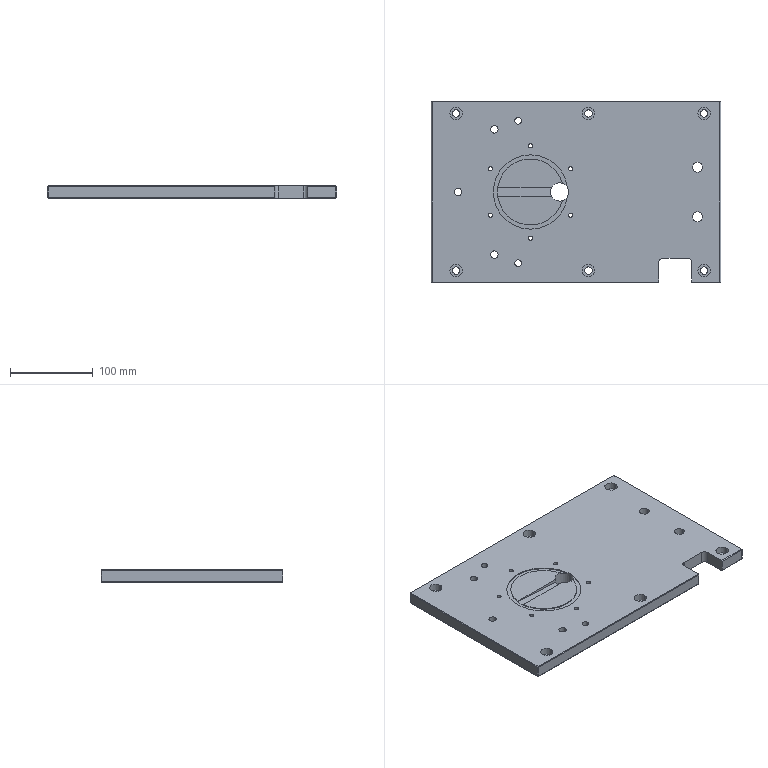Component | SolidWorks | ZN-A-008-1 | 1 solid | 110 faces | box 350 x 220 x 15 mm | volume 1103345 mm3 | cylinder 63 | plane 47 | commonest cylinder face diameters 15 x18 9 x18 5 x12 12 x4 8 x4 22 x2 80 x2 10 x2
build123d program:
from build123d import *

# Parameters (mm, degrees)
SKETCH1_W                                       = 350
SKETCH1_H                                       = 220
BOSS_EXTRUDE1_DEPTH                             = 15
F_8_0_8_DIAMETER_HOLE1_D                        = 8
F_8_0_8_DIAMETER_HOLE1_DEPTH                    = 15
F_8_0_8_DIAMETER_HOLE1_TIP                      = 2.403
M8_HEX_SOCKET_HEAD_CAP_SCREW_CBORE1_D           = 9
M8_HEX_SOCKET_HEAD_CAP_SCREW_CBORE1_CBORE_D     = 15
M8_HEX_SOCKET_HEAD_CAP_SCREW_CBORE1_CBORE_DEPTH = 8.6
M12_TAPPED_HOLE1_D                              = 12
M12_TAPPED_HOLE1_DEPTH                          = 29.25
M12_TAPPED_HOLE1_TIP                            = 3.605
M8_HEX_SOCKET_HEAD_CAP_SCREW_CBORE2_D           = 9
M8_HEX_SOCKET_HEAD_CAP_SCREW_CBORE2_CBORE_D     = 15
M8_HEX_SOCKET_HEAD_CAP_SCREW_CBORE2_CBORE_DEPTH = 8.6
CUT_EXTRUDE2_DEPTH                              = 50
CHAMFER2_SIZE                                   = 1
SKETCH12_R                                      = 11
CUT_EXTRUDE3_DEPTH                              = 90
SKETCH14_R                                      = 45
SKETCH14_R_2                                    = 40
CUT_EXTRUDE7_DEPTH                              = 1
CUT_EXTRUDE6_DEPTH                              = 5
CUT_EXTRUDE6_DEPTH_BACK                         = 5
M6_TAPPED_HOLE1_D                               = 5
M6_TAPPED_HOLE1_DEPTH                           = 15
M6_TAPPED_HOLE1_TIP                             = 1.502


with BuildPart() as part:
    # Sketch1 → Boss-Extrude1 (new body)
    with BuildSketch(Plane.XY):
        with Locations((473.392, 232.499)):
            Rectangle(SKETCH1_W, SKETCH1_H)
    extrude(amount=BOSS_EXTRUDE1_DEPTH)

    # 8.0 _8_ Diameter Hole1
    with Locations(Plane(origin=(0, 0, 0), x_dir=(-1, 0, 0), z_dir=(0, 0, -1))):
        with Locations((-403.392, 146.295), (-403.392, 318.704)):
            Hole(F_8_0_8_DIAMETER_HOLE1_D / 2, depth=F_8_0_8_DIAMETER_HOLE1_DEPTH)
            with Locations((0, 0, -(F_8_0_8_DIAMETER_HOLE1_DEPTH + F_8_0_8_DIAMETER_HOLE1_TIP / 2))):  # 118° drill point
                Cone(0, F_8_0_8_DIAMETER_HOLE1_D / 2, F_8_0_8_DIAMETER_HOLE1_TIP, mode=Mode.SUBTRACT)

    # M8 Hex Socket Head Cap Screw CBORE1 (through all)
    with Locations(Plane(origin=(0, 0, 0), x_dir=(-1, 0, 0), z_dir=(0, 0, -1))):
        with Locations((-374.642, 156.722), (-330.892, 232.499), (-374.642, 308.277)):
            CounterBoreHole(M8_HEX_SOCKET_HEAD_CAP_SCREW_CBORE1_D / 2, M8_HEX_SOCKET_HEAD_CAP_SCREW_CBORE1_CBORE_D / 2, M8_HEX_SOCKET_HEAD_CAP_SCREW_CBORE1_CBORE_DEPTH)

    # M12 Tapped Hole1
    with Locations(Plane.XY.offset(15)):
        with Locations((620.392, 262.499), (620.392, 202.499)):
            Hole(M12_TAPPED_HOLE1_D / 2, depth=M12_TAPPED_HOLE1_DEPTH)
            with Locations((0, 0, -(M12_TAPPED_HOLE1_DEPTH + M12_TAPPED_HOLE1_TIP / 2))):  # 118° drill point
                Cone(0, M12_TAPPED_HOLE1_D / 2, M12_TAPPED_HOLE1_TIP, mode=Mode.SUBTRACT)

    # M8 Hex Socket Head Cap Screw CBORE2 (through all)
    with Locations(Plane.XY.offset(15)):
        with Locations((328.392, 327.499), (628.392, 327.499), (488.392, 327.499), (328.392, 137.499), (628.392, 137.499), (488.392, 137.499)):
            CounterBoreHole(M8_HEX_SOCKET_HEAD_CAP_SCREW_CBORE2_D / 2, M8_HEX_SOCKET_HEAD_CAP_SCREW_CBORE2_CBORE_D / 2, M8_HEX_SOCKET_HEAD_CAP_SCREW_CBORE2_CBORE_DEPTH)

    # Sketch11 → Cut-Extrude2 (cut)
    with BuildSketch(Plane.XY.offset(15)):
        with BuildLine():
            Line((573.392, 101.608), (613.392, 101.608))
            Line((613.392, 101.608), (613.392, 147.499))
            ThreePointArc((613.392, 147.499), (611.927, 151.035), (608.392, 152.499))
            Line((608.392, 152.499), (578.392, 152.499))
            ThreePointArc((578.392, 152.499), (574.856, 151.035), (573.392, 147.499))
            Line((573.392, 147.499), (573.392, 101.608))
        make_face()
    extrude(amount=-CUT_EXTRUDE2_DEPTH, mode=Mode.SUBTRACT)

    # Chamfer2
    chamfer2_edges = [part.edges().sort_by_distance(p)[0] for p in [
        (648.392, 232.499, 15),
        (630.892, 122.499, 0),
        (630.892, 122.499, 15),
        (473.392, 342.499, 15),
        (298.392, 232.499, 15),
        (473.392, 342.499, 0),
        (648.392, 232.499, 0),
        (435.892, 122.499, 0),
        (298.392, 232.499, 0),
        (435.892, 122.499, 15),
        (298.392, 342.499, 7.5),
        (648.392, 342.499, 7.5),
        (648.392, 122.499, 7.5),
        (298.392, 122.499, 7.5),
    ]]
    chamfer(chamfer2_edges, length=CHAMFER2_SIZE)

    # Sketch12 → Cut-Extrude3 (cut)
    with BuildSketch(Plane(origin=(0, 0, 0), x_dir=(-1, 0, 0), z_dir=(0, 0, -1))):
        with Locations((-453.392, 232.499)):
            Circle(SKETCH12_R)
    extrude(amount=-CUT_EXTRUDE3_DEPTH, mode=Mode.SUBTRACT)

    # Sketch14 → Cut-Extrude7 (cut)
    with BuildSketch(Plane.XY.offset(15)):
        with Locations((418.392, 232.499)):
            Circle(SKETCH14_R)
        with Locations((418.392, 232.499)):
            Circle(SKETCH14_R_2, mode=Mode.SUBTRACT)
    extrude(amount=-CUT_EXTRUDE7_DEPTH, mode=Mode.SUBTRACT)

    # Sketch13 → Cut-Extrude6 (cut, two sides: drawn at the far end of the back side and taken through both)
    with BuildSketch(Plane(origin=(0, 232.499, 0), x_dir=(1, 0, 0), z_dir=(0, 1, 0)).offset(-CUT_EXTRUDE6_DEPTH_BACK)):
        Polygon((378.392, -14), (448.392, -10.331), (448.392, -15), (378.392, -15), align=None)
    extrude(amount=CUT_EXTRUDE6_DEPTH + CUT_EXTRUDE6_DEPTH_BACK, mode=Mode.SUBTRACT)

    # M6 Tapped Hole1
    with Locations(Plane.XY.offset(15)):
        with Locations((369.894, 260.499), (418.392, 288.499), (369.894, 204.499), (418.392, 176.499), (466.889, 204.499), (466.889, 260.499)):
            Hole(M6_TAPPED_HOLE1_D / 2, depth=M6_TAPPED_HOLE1_DEPTH)
            with Locations((0, 0, -(M6_TAPPED_HOLE1_DEPTH + M6_TAPPED_HOLE1_TIP / 2))):  # 118° drill point
                Cone(0, M6_TAPPED_HOLE1_D / 2, M6_TAPPED_HOLE1_TIP, mode=Mode.SUBTRACT)


solid = part.part